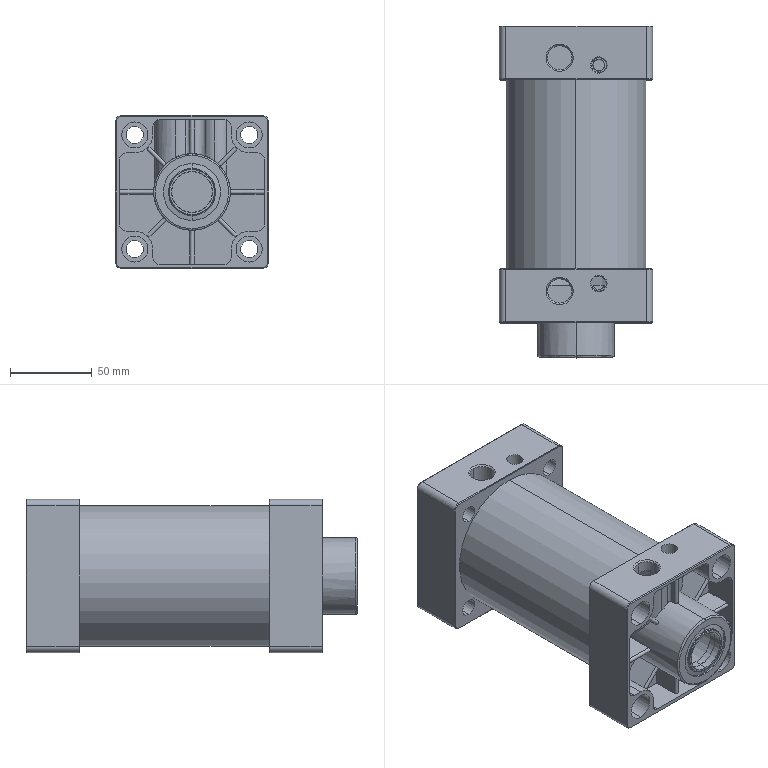Component | SolidWorks | SC-80x75(000)-1_1-1 | 1 solid | 298 faces | volume 369259 mm3 | cylinder 132 | plane 128 | cone 30 | spline 8 | commonest cylinder face diameters 8 x27 16 x21 2.5 x18 10.5 x16 22 x8 26 x5 10.1 x4 14.95 x4